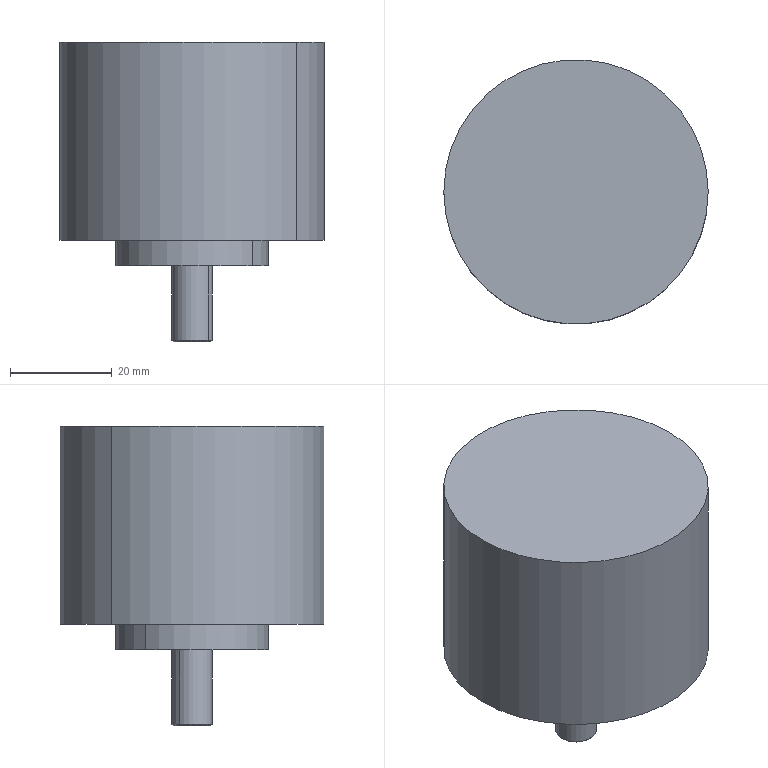Component | SolidWorks | LD101-02-RotaryEncoder-0002-2-2 | 1 solid | 24 faces | box 52 x 52 x 59 mm | volume 86983 mm3 | cylinder 12 | cone 8 | plane 4 | commonest cylinder face diameters 2.5 x6 8 x2 30 x2 52 x2 | material AL6061
STEP:
#1=COLOUR_RGB('',0.7922,0.8196,0.9333);
#2=FILL_AREA_STYLE_COLOUR('',#1);
#3=FILL_AREA_STYLE('',(#2));
#4=SURFACE_STYLE_FILL_AREA(#3);
#5=SURFACE_SIDE_STYLE('',(#4));
#6=SURFACE_STYLE_USAGE(.BOTH.,#5);
#7=PRESENTATION_STYLE_ASSIGNMENT((#6));
#8=CARTESIAN_POINT('',(5.132,-7.919,13.573));
#9=VERTEX_POINT('',#8);
#10=CARTESIAN_POINT('',(5.054,-7.859,13.573));
#11=VERTEX_POINT('',#10);
#12=CARTESIAN_POINT('',(5.093,-7.889,13.573));
#13=DIRECTION('',(0.,0.,-1.));
#14=DIRECTION('',(-0.7932,0.609,0.));
#15=AXIS2_PLACEMENT_3D('',#12,#13,#14);
#16=CIRCLE('',#15,0.04921);
#17=EDGE_CURVE('',#9,#11,#16,.T.);
#18=ORIENTED_EDGE('',*,*,#17,.F.);
#19=CARTESIAN_POINT('',(5.132,-7.919,13.238));
#20=VERTEX_POINT('',#19);
#21=CARTESIAN_POINT('',(5.132,-7.919,13.238));
#22=DIRECTION('',(0.,0.,-1.));
#23=VECTOR('',#22,39.37);
#24=LINE('',#21,#23);
#25=EDGE_CURVE('',#9,#20,#24,.T.);
#26=ORIENTED_EDGE('',*,*,#25,.T.);
#27=CARTESIAN_POINT('',(5.054,-7.859,13.238));
#28=VERTEX_POINT('',#27);
#29=CARTESIAN_POINT('',(5.093,-7.889,13.238));
#30=DIRECTION('',(0.,0.,-1.));
#31=DIRECTION('',(-0.7932,0.609,0.));
#32=AXIS2_PLACEMENT_3D('',#29,#30,#31);
#33=CIRCLE('',#32,0.04921);
#34=EDGE_CURVE('',#20,#28,#33,.T.);
#35=ORIENTED_EDGE('',*,*,#34,.T.);
#36=CARTESIAN_POINT('',(5.054,-7.859,13.238));
#37=DIRECTION('',(0.,0.,-1.));
#38=VECTOR('',#37,39.37);
#39=LINE('',#36,#38);
#40=EDGE_CURVE('',#11,#28,#39,.T.);
#41=ORIENTED_EDGE('',*,*,#40,.F.);
#42=EDGE_LOOP('',(#18,#26,#35,#41));
#43=FACE_OUTER_BOUND('',#42,.T.);
#44=CARTESIAN_POINT('',(5.093,-7.889,13.238));
#45=DIRECTION('',(0.,0.,-1.));
#46=DIRECTION('',(-0.7932,0.609,0.));
#47=AXIS2_PLACEMENT_3D('',#44,#45,#46);
#48=CYLINDRICAL_SURFACE('',#47,0.04921);
#49=ADVANCED_FACE('',(#43),#48,.F.);
#50=CARTESIAN_POINT('',(5.093,-7.889,13.603));
#51=VERTEX_POINT('',#50);
#52=CARTESIAN_POINT('',(5.054,-7.859,13.573));
#53=DIRECTION('',(-0.6799,0.522,-0.515));
#54=VECTOR('',#53,39.37);
#55=LINE('',#52,#54);
#56=EDGE_CURVE('',#51,#11,#55,.T.);
#57=ORIENTED_EDGE('',*,*,#56,.F.);
#58=CARTESIAN_POINT('',(5.132,-7.919,13.573));
#59=DIRECTION('',(0.6799,-0.522,-0.515));
#60=VECTOR('',#59,39.37);
#61=LINE('',#58,#60);
#62=EDGE_CURVE('',#51,#9,#61,.T.);
#63=ORIENTED_EDGE('',*,*,#62,.T.);
#64=ORIENTED_EDGE('',*,*,#17,.T.);
#65=EDGE_LOOP('',(#57,#63,#64));
#66=FACE_OUTER_BOUND('',#65,.T.);
#67=CARTESIAN_POINT('',(5.093,-7.889,13.573));
#68=DIRECTION('',(0.,0.,-1.));
#69=DIRECTION('',(-0.7932,0.609,0.));
#70=AXIS2_PLACEMENT_3D('',#67,#68,#69);
#71=CONICAL_SURFACE('',#70,0.04921,1.03);
#72=ADVANCED_FACE('',(#66),#71,.F.);
#73=CARTESIAN_POINT('',(4.05,-7.088,13.573));
#74=VERTEX_POINT('',#73);
#75=CARTESIAN_POINT('',(3.972,-7.028,13.573));
#76=VERTEX_POINT('',#75);
#77=CARTESIAN_POINT('',(4.011,-7.058,13.573));
#78=DIRECTION('',(0.,0.,-1.));
#79=DIRECTION('',(-0.7932,0.609,0.));
#80=AXIS2_PLACEMENT_3D('',#77,#78,#79);
#81=CIRCLE('',#80,0.04921);
#82=EDGE_CURVE('',#74,#76,#81,.T.);
#83=ORIENTED_EDGE('',*,*,#82,.F.);
#84=CARTESIAN_POINT('',(4.05,-7.088,13.238));
#85=VERTEX_POINT('',#84);
#86=CARTESIAN_POINT('',(4.05,-7.088,13.238));
#87=DIRECTION('',(0.,0.,-1.));
#88=VECTOR('',#87,39.37);
#89=LINE('',#86,#88);
#90=EDGE_CURVE('',#74,#85,#89,.T.);
#91=ORIENTED_EDGE('',*,*,#90,.T.);
#92=CARTESIAN_POINT('',(3.972,-7.028,13.238));
#93=VERTEX_POINT('',#92);
#94=CARTESIAN_POINT('',(4.011,-7.058,13.238));
#95=DIRECTION('',(0.,0.,-1.));
#96=DIRECTION('',(-0.7932,0.609,0.));
#97=AXIS2_PLACEMENT_3D('',#94,#95,#96);
#98=CIRCLE('',#97,0.04921);
#99=EDGE_CURVE('',#85,#93,#98,.T.);
#100=ORIENTED_EDGE('',*,*,#99,.T.);
#101=CARTESIAN_POINT('',(3.972,-7.028,13.238));
#102=DIRECTION('',(0.,0.,-1.));
#103=VECTOR('',#102,39.37);
#104=LINE('',#101,#103);
#105=EDGE_CURVE('',#76,#93,#104,.T.);
#106=ORIENTED_EDGE('',*,*,#105,.F.);
#107=EDGE_LOOP('',(#83,#91,#100,#106));
#108=FACE_OUTER_BOUND('',#107,.T.);
#109=CARTESIAN_POINT('',(4.011,-7.058,13.238));
#110=DIRECTION('',(0.,0.,-1.));
#111=DIRECTION('',(-0.7932,0.609,0.));
#112=AXIS2_PLACEMENT_3D('',#109,#110,#111);
#113=CYLINDRICAL_SURFACE('',#112,0.04921);
#114=ADVANCED_FACE('',(#108),#113,.F.);
#115=CARTESIAN_POINT('',(4.011,-7.058,13.603));
#116=VERTEX_POINT('',#115);
#117=CARTESIAN_POINT('',(3.972,-7.028,13.573));
#118=DIRECTION('',(-0.6799,0.522,-0.515));
#119=VECTOR('',#118,39.37);
#120=LINE('',#117,#119);
#121=EDGE_CURVE('',#116,#76,#120,.T.);
#122=ORIENTED_EDGE('',*,*,#121,.F.);
#123=CARTESIAN_POINT('',(4.05,-7.088,13.573));
#124=DIRECTION('',(0.6799,-0.522,-0.515));
#125=VECTOR('',#124,39.37);
#126=LINE('',#123,#125);
#127=EDGE_CURVE('',#116,#74,#126,.T.);
#128=ORIENTED_EDGE('',*,*,#127,.T.);
#129=ORIENTED_EDGE('',*,*,#82,.T.);
#130=EDGE_LOOP('',(#122,#128,#129));
#131=FACE_OUTER_BOUND('',#130,.T.);
#132=CARTESIAN_POINT('',(4.011,-7.058,13.573));
#133=DIRECTION('',(0.,0.,-1.));
#134=DIRECTION('',(-0.7932,0.609,0.));
#135=AXIS2_PLACEMENT_3D('',#132,#133,#134);
#136=CONICAL_SURFACE('',#135,0.04921,1.03);
#137=ADVANCED_FACE('',(#131),#136,.F.);
#138=CARTESIAN_POINT('',(5.31,-6.567,13.573));
#139=VERTEX_POINT('',#138);
#140=CARTESIAN_POINT('',(5.232,-6.507,13.573));
#141=VERTEX_POINT('',#140);
#142=CARTESIAN_POINT('',(5.271,-6.537,13.573));
#143=DIRECTION('',(0.,0.,-1.));
#144=DIRECTION('',(-0.7932,0.609,0.));
#145=AXIS2_PLACEMENT_3D('',#142,#143,#144);
#146=CIRCLE('',#145,0.04921);
#147=EDGE_CURVE('',#139,#141,#146,.T.);
#148=ORIENTED_EDGE('',*,*,#147,.F.);
#149=CARTESIAN_POINT('',(5.31,-6.567,13.238));
#150=VERTEX_POINT('',#149);
#151=CARTESIAN_POINT('',(5.31,-6.567,13.238));
#152=DIRECTION('',(0.,0.,-1.));
#153=VECTOR('',#152,39.37);
#154=LINE('',#151,#153);
#155=EDGE_CURVE('',#139,#150,#154,.T.);
#156=ORIENTED_EDGE('',*,*,#155,.T.);
#157=CARTESIAN_POINT('',(5.232,-6.507,13.238));
#158=VERTEX_POINT('',#157);
#159=CARTESIAN_POINT('',(5.271,-6.537,13.238));
#160=DIRECTION('',(0.,0.,-1.));
#161=DIRECTION('',(-0.7932,0.609,0.));
#162=AXIS2_PLACEMENT_3D('',#159,#160,#161);
#163=CIRCLE('',#162,0.04921);
#164=EDGE_CURVE('',#150,#158,#163,.T.);
#165=ORIENTED_EDGE('',*,*,#164,.T.);
#166=CARTESIAN_POINT('',(5.232,-6.507,13.238));
#167=DIRECTION('',(0.,0.,-1.));
#168=VECTOR('',#167,39.37);
#169=LINE('',#166,#168);
#170=EDGE_CURVE('',#141,#158,#169,.T.);
#171=ORIENTED_EDGE('',*,*,#170,.F.);
#172=EDGE_LOOP('',(#148,#156,#165,#171));
#173=FACE_OUTER_BOUND('',#172,.T.);
#174=CARTESIAN_POINT('',(5.271,-6.537,13.238));
#175=DIRECTION('',(0.,0.,-1.));
#176=DIRECTION('',(-0.7932,0.609,0.));
#177=AXIS2_PLACEMENT_3D('',#174,#175,#176);
#178=CYLINDRICAL_SURFACE('',#177,0.04921);
#179=ADVANCED_FACE('',(#173),#178,.F.);
#180=CARTESIAN_POINT('',(5.271,-6.537,13.603));
#181=VERTEX_POINT('',#180);
#182=CARTESIAN_POINT('',(5.232,-6.507,13.573));
#183=DIRECTION('',(-0.6799,0.522,-0.515));
#184=VECTOR('',#183,39.37);
#185=LINE('',#182,#184);
#186=EDGE_CURVE('',#181,#141,#185,.T.);
#187=ORIENTED_EDGE('',*,*,#186,.F.);
#188=CARTESIAN_POINT('',(5.31,-6.567,13.573));
#189=DIRECTION('',(0.6799,-0.522,-0.515));
#190=VECTOR('',#189,39.37);
#191=LINE('',#188,#190);
#192=EDGE_CURVE('',#181,#139,#191,.T.);
#193=ORIENTED_EDGE('',*,*,#192,.T.);
#194=ORIENTED_EDGE('',*,*,#147,.T.);
#195=EDGE_LOOP('',(#187,#193,#194));
#196=FACE_OUTER_BOUND('',#195,.T.);
#197=CARTESIAN_POINT('',(5.271,-6.537,13.573));
#198=DIRECTION('',(0.,0.,-1.));
#199=DIRECTION('',(-0.7932,0.609,0.));
#200=AXIS2_PLACEMENT_3D('',#197,#198,#199);
#201=CONICAL_SURFACE('',#200,0.04921,1.03);
#202=ADVANCED_FACE('',(#196),#201,.F.);
#203=CARTESIAN_POINT('',(4.676,-7.073,12.451));
#204=VERTEX_POINT('',#203);
#205=CARTESIAN_POINT('',(4.907,-7.25,12.451));
#206=VERTEX_POINT('',#205);
#207=CARTESIAN_POINT('',(4.792,-7.161,12.451));
#208=DIRECTION('',(0.,0.,-1.));
#209=DIRECTION('',(-0.7932,0.609,0.));
#210=AXIS2_PLACEMENT_3D('',#207,#208,#209);
#211=CIRCLE('',#210,0.1457);
#212=EDGE_CURVE('',#204,#206,#211,.T.);
#213=ORIENTED_EDGE('',*,*,#212,.F.);
#214=CARTESIAN_POINT('',(4.667,-7.065,12.463));
#215=VERTEX_POINT('',#214);
#216=CARTESIAN_POINT('',(4.676,-7.073,12.451));
#217=DIRECTION('',(-0.5609,0.4306,0.7071));
#218=VECTOR('',#217,39.37);
#219=LINE('',#216,#218);
#220=EDGE_CURVE('',#204,#215,#219,.T.);
#221=ORIENTED_EDGE('',*,*,#220,.T.);
#222=CARTESIAN_POINT('',(4.917,-7.257,12.463));
#223=VERTEX_POINT('',#222);
#224=CARTESIAN_POINT('',(4.792,-7.161,12.463));
#225=DIRECTION('',(0.,0.,1.));
#226=DIRECTION('',(-0.7932,0.609,0.));
#227=AXIS2_PLACEMENT_3D('',#224,#225,#226);
#228=CIRCLE('',#227,0.1575);
#229=EDGE_CURVE('',#223,#215,#228,.T.);
#230=ORIENTED_EDGE('',*,*,#229,.F.);
#231=CARTESIAN_POINT('',(4.907,-7.25,12.451));
#232=DIRECTION('',(0.5609,-0.4306,0.7071));
#233=VECTOR('',#232,39.37);
#234=LINE('',#231,#233);
#235=EDGE_CURVE('',#206,#223,#234,.T.);
#236=ORIENTED_EDGE('',*,*,#235,.F.);
#237=EDGE_LOOP('',(#213,#221,#230,#236));
#238=FACE_OUTER_BOUND('',#237,.T.);
#239=CARTESIAN_POINT('',(4.792,-7.161,12.451));
#240=DIRECTION('',(0.,0.,1.));
#241=DIRECTION('',(0.7932,-0.609,0.));
#242=AXIS2_PLACEMENT_3D('',#239,#240,#241);
#243=CONICAL_SURFACE('',#242,0.1457,0.7854);
#244=ADVANCED_FACE('',(#238),#243,.T.);
#245=ORIENTED_EDGE('',*,*,#229,.T.);
#246=CARTESIAN_POINT('',(4.667,-7.065,13.042));
#247=VERTEX_POINT('',#246);
#248=CARTESIAN_POINT('',(4.667,-7.065,12.451));
#249=DIRECTION('',(0.,0.,1.));
#250=VECTOR('',#249,39.37);
#251=LINE('',#248,#250);
#252=EDGE_CURVE('',#215,#247,#251,.T.);
#253=ORIENTED_EDGE('',*,*,#252,.T.);
#254=CARTESIAN_POINT('',(4.917,-7.257,13.042));
#255=VERTEX_POINT('',#254);
#256=CARTESIAN_POINT('',(4.792,-7.161,13.042));
#257=DIRECTION('',(0.,0.,-1.));
#258=DIRECTION('',(-0.7932,0.609,0.));
#259=AXIS2_PLACEMENT_3D('',#256,#257,#258);
#260=CIRCLE('',#259,0.1575);
#261=EDGE_CURVE('',#247,#255,#260,.T.);
#262=ORIENTED_EDGE('',*,*,#261,.T.);
#263=CARTESIAN_POINT('',(4.917,-7.257,12.451));
#264=DIRECTION('',(0.,0.,1.));
#265=VECTOR('',#264,39.37);
#266=LINE('',#263,#265);
#267=EDGE_CURVE('',#223,#255,#266,.T.);
#268=ORIENTED_EDGE('',*,*,#267,.F.);
#269=EDGE_LOOP('',(#245,#253,#262,#268));
#270=FACE_OUTER_BOUND('',#269,.T.);
#271=CARTESIAN_POINT('',(4.792,-7.161,12.451));
#272=DIRECTION('',(0.,0.,1.));
#273=DIRECTION('',(0.7932,-0.609,0.));
#274=AXIS2_PLACEMENT_3D('',#271,#272,#273);
#275=CYLINDRICAL_SURFACE('',#274,0.1575);
#276=ADVANCED_FACE('',(#270),#275,.T.);
#277=CARTESIAN_POINT('',(4.323,-6.802,13.042));
#278=VERTEX_POINT('',#277);
#279=CARTESIAN_POINT('',(5.26,-7.521,13.042));
#280=VERTEX_POINT('',#279);
#281=CARTESIAN_POINT('',(4.792,-7.161,13.042));
#282=DIRECTION('',(0.,0.,-1.));
#283=DIRECTION('',(-0.7932,0.609,0.));
#284=AXIS2_PLACEMENT_3D('',#281,#282,#283);
#285=CIRCLE('',#284,0.5906);
#286=EDGE_CURVE('',#278,#280,#285,.T.);
#287=ORIENTED_EDGE('',*,*,#286,.F.);
#288=CARTESIAN_POINT('',(4.323,-6.802,13.238));
#289=VERTEX_POINT('',#288);
#290=CARTESIAN_POINT('',(4.323,-6.802,13.042));
#291=DIRECTION('',(0.,0.,1.));
#292=VECTOR('',#291,39.37);
#293=LINE('',#290,#292);
#294=EDGE_CURVE('',#278,#289,#293,.T.);
#295=ORIENTED_EDGE('',*,*,#294,.T.);
#296=CARTESIAN_POINT('',(5.26,-7.521,13.238));
#297=VERTEX_POINT('',#296);
#298=CARTESIAN_POINT('',(4.792,-7.161,13.238));
#299=DIRECTION('',(0.,0.,-1.));
#300=DIRECTION('',(-0.7932,0.609,0.));
#301=AXIS2_PLACEMENT_3D('',#298,#299,#300);
#302=CIRCLE('',#301,0.5906);
#303=EDGE_CURVE('',#289,#297,#302,.T.);
#304=ORIENTED_EDGE('',*,*,#303,.T.);
#305=CARTESIAN_POINT('',(5.26,-7.521,13.042));
#306=DIRECTION('',(0.,0.,1.));
#307=VECTOR('',#306,39.37);
#308=LINE('',#305,#307);
#309=EDGE_CURVE('',#280,#297,#308,.T.);
#310=ORIENTED_EDGE('',*,*,#309,.F.);
#311=EDGE_LOOP('',(#287,#295,#304,#310));
#312=FACE_OUTER_BOUND('',#311,.T.);
#313=CARTESIAN_POINT('',(4.792,-7.161,13.042));
#314=DIRECTION('',(0.,0.,1.));
#315=DIRECTION('',(0.7932,-0.609,0.));
#316=AXIS2_PLACEMENT_3D('',#313,#314,#315);
#317=CYLINDRICAL_SURFACE('',#316,0.5906);
#318=ADVANCED_FACE('',(#312),#317,.T.);
#319=CARTESIAN_POINT('',(3.98,-6.538,14.774));
#320=VERTEX_POINT('',#319);
#321=CARTESIAN_POINT('',(5.604,-7.785,14.774));
#322=VERTEX_POINT('',#321);
#323=CARTESIAN_POINT('',(4.792,-7.161,14.774));
#324=DIRECTION('',(0.,0.,-1.));
#325=DIRECTION('',(-0.7932,0.609,0.));
#326=AXIS2_PLACEMENT_3D('',#323,#324,#325);
#327=CIRCLE('',#326,1.024);
#328=EDGE_CURVE('',#320,#322,#327,.T.);
#329=ORIENTED_EDGE('',*,*,#328,.T.);
#330=CARTESIAN_POINT('',(5.604,-7.785,13.238));
#331=VERTEX_POINT('',#330);
#332=CARTESIAN_POINT('',(5.604,-7.785,14.774));
#333=DIRECTION('',(0.,0.,-1.));
#334=VECTOR('',#333,39.37);
#335=LINE('',#332,#334);
#336=EDGE_CURVE('',#322,#331,#335,.T.);
#337=ORIENTED_EDGE('',*,*,#336,.T.);
#338=CARTESIAN_POINT('',(3.98,-6.538,13.238));
#339=VERTEX_POINT('',#338);
#340=CARTESIAN_POINT('',(4.792,-7.161,13.238));
#341=DIRECTION('',(0.,0.,-1.));
#342=DIRECTION('',(-0.7932,0.609,0.));
#343=AXIS2_PLACEMENT_3D('',#340,#341,#342);
#344=CIRCLE('',#343,1.024);
#345=EDGE_CURVE('',#339,#331,#344,.T.);
#346=ORIENTED_EDGE('',*,*,#345,.F.);
#347=CARTESIAN_POINT('',(3.98,-6.538,14.774));
#348=DIRECTION('',(0.,0.,-1.));
#349=VECTOR('',#348,39.37);
#350=LINE('',#347,#349);
#351=EDGE_CURVE('',#320,#339,#350,.T.);
#352=ORIENTED_EDGE('',*,*,#351,.F.);
#353=EDGE_LOOP('',(#329,#337,#346,#352));
#354=FACE_OUTER_BOUND('',#353,.T.);
#355=CARTESIAN_POINT('',(4.792,-7.161,14.774));
#356=DIRECTION('',(0.,0.,-1.));
#357=DIRECTION('',(-0.7932,0.609,0.));
#358=AXIS2_PLACEMENT_3D('',#355,#356,#357);
#359=CYLINDRICAL_SURFACE('',#358,1.024);
#360=ADVANCED_FACE('',(#354),#359,.T.);
#361=CARTESIAN_POINT('',(4.792,-7.161,13.042));
#362=DIRECTION('',(0.,0.,-1.));
#363=DIRECTION('',(-0.7932,0.609,0.));
#364=AXIS2_PLACEMENT_3D('',#361,#362,#363);
#365=CIRCLE('',#364,0.5906);
#366=EDGE_CURVE('',#280,#278,#365,.T.);
#367=ORIENTED_EDGE('',*,*,#366,.T.);
#368=ORIENTED_EDGE('',*,*,#286,.T.);
#369=EDGE_LOOP('',(#367,#368));
#370=FACE_OUTER_BOUND('',#369,.T.);
#371=CARTESIAN_POINT('',(4.792,-7.161,13.042));
#372=DIRECTION('',(0.,0.,-1.));
#373=DIRECTION('',(-0.7932,0.609,0.));
#374=AXIS2_PLACEMENT_3D('',#371,#372,#373);
#375=CIRCLE('',#374,0.1575);
#376=EDGE_CURVE('',#255,#247,#375,.T.);
#377=ORIENTED_EDGE('',*,*,#376,.F.);
#378=ORIENTED_EDGE('',*,*,#261,.F.);
#379=EDGE_LOOP('',(#377,#378));
#380=FACE_BOUND('',#379,.T.);
#381=CARTESIAN_POINT('',(4.792,-7.161,13.042));
#382=DIRECTION('',(0.,0.,-1.));
#383=DIRECTION('',(-0.7932,0.609,0.));
#384=AXIS2_PLACEMENT_3D('',#381,#382,#383);
#385=PLANE('',#384);
#386=ADVANCED_FACE('',(#370,#380),#385,.T.);
#387=CARTESIAN_POINT('',(5.093,-7.889,13.238));
#388=DIRECTION('',(0.,0.,-1.));
#389=DIRECTION('',(-0.7932,0.609,0.));
#390=AXIS2_PLACEMENT_3D('',#387,#388,#389);
#391=CIRCLE('',#390,0.04921);
#392=EDGE_CURVE('',#28,#20,#391,.T.);
#393=ORIENTED_EDGE('',*,*,#392,.F.);
#394=ORIENTED_EDGE('',*,*,#34,.F.);
#395=EDGE_LOOP('',(#393,#394));
#396=FACE_BOUND('',#395,.T.);
#397=CARTESIAN_POINT('',(4.011,-7.058,13.238));
#398=DIRECTION('',(0.,0.,-1.));
#399=DIRECTION('',(-0.7932,0.609,0.));
#400=AXIS2_PLACEMENT_3D('',#397,#398,#399);
#401=CIRCLE('',#400,0.04921);
#402=EDGE_CURVE('',#93,#85,#401,.T.);
#403=ORIENTED_EDGE('',*,*,#402,.F.);
#404=ORIENTED_EDGE('',*,*,#99,.F.);
#405=EDGE_LOOP('',(#403,#404));
#406=FACE_BOUND('',#405,.T.);
#407=CARTESIAN_POINT('',(5.271,-6.537,13.238));
#408=DIRECTION('',(0.,0.,-1.));
#409=DIRECTION('',(-0.7932,0.609,0.));
#410=AXIS2_PLACEMENT_3D('',#407,#408,#409);
#411=CIRCLE('',#410,0.04921);
#412=EDGE_CURVE('',#158,#150,#411,.T.);
#413=ORIENTED_EDGE('',*,*,#412,.F.);
#414=ORIENTED_EDGE('',*,*,#164,.F.);
#415=EDGE_LOOP('',(#413,#414));
#416=FACE_BOUND('',#415,.T.);
#417=ORIENTED_EDGE('',*,*,#345,.T.);
#418=CARTESIAN_POINT('',(4.792,-7.161,13.238));
#419=DIRECTION('',(0.,0.,-1.));
#420=DIRECTION('',(-0.7932,0.609,0.));
#421=AXIS2_PLACEMENT_3D('',#418,#419,#420);
#422=CIRCLE('',#421,1.024);
#423=EDGE_CURVE('',#331,#339,#422,.T.);
#424=ORIENTED_EDGE('',*,*,#423,.T.);
#425=EDGE_LOOP('',(#417,#424));
#426=FACE_OUTER_BOUND('',#425,.T.);
#427=CARTESIAN_POINT('',(4.792,-7.161,13.238));
#428=DIRECTION('',(0.,0.,-1.));
#429=DIRECTION('',(-0.7932,0.609,0.));
#430=AXIS2_PLACEMENT_3D('',#427,#428,#429);
#431=CIRCLE('',#430,0.5906);
#432=EDGE_CURVE('',#297,#289,#431,.T.);
#433=ORIENTED_EDGE('',*,*,#432,.F.);
#434=ORIENTED_EDGE('',*,*,#303,.F.);
#435=EDGE_LOOP('',(#433,#434));
#436=FACE_BOUND('',#435,.T.);
#437=CARTESIAN_POINT('',(4.792,-7.161,13.238));
#438=DIRECTION('',(0.,0.,-1.));
#439=DIRECTION('',(-0.7932,0.609,0.));
#440=AXIS2_PLACEMENT_3D('',#437,#438,#439);
#441=PLANE('',#440);
#442=ADVANCED_FACE('',(#396,#406,#416,#426,#436),#441,.T.);
#443=ORIENTED_EDGE('',*,*,#336,.F.);
#444=CARTESIAN_POINT('',(4.792,-7.161,14.774));
#445=DIRECTION('',(0.,0.,-1.));
#446=DIRECTION('',(-0.7932,0.609,0.));
#447=AXIS2_PLACEMENT_3D('',#444,#445,#446);
#448=CIRCLE('',#447,1.024);
#449=EDGE_CURVE('',#322,#320,#448,.T.);
#450=ORIENTED_EDGE('',*,*,#449,.T.);
#451=ORIENTED_EDGE('',*,*,#351,.T.);
#452=ORIENTED_EDGE('',*,*,#423,.F.);
#453=EDGE_LOOP('',(#443,#450,#451,#452));
#454=FACE_OUTER_BOUND('',#453,.T.);
#455=CARTESIAN_POINT('',(4.792,-7.161,14.774));
#456=DIRECTION('',(0.,0.,-1.));
#457=DIRECTION('',(-0.7932,0.609,0.));
#458=AXIS2_PLACEMENT_3D('',#455,#456,#457);
#459=CYLINDRICAL_SURFACE('',#458,1.024);
#460=ADVANCED_FACE('',(#454),#459,.T.);
#461=ORIENTED_EDGE('',*,*,#328,.F.);
#462=ORIENTED_EDGE('',*,*,#449,.F.);
#463=EDGE_LOOP('',(#461,#462));
#464=FACE_OUTER_BOUND('',#463,.T.);
#465=CARTESIAN_POINT('',(4.792,-7.161,14.774));
#466=DIRECTION('',(0.,0.,-1.));
#467=DIRECTION('',(-0.7932,0.609,0.));
#468=AXIS2_PLACEMENT_3D('',#465,#466,#467);
#469=PLANE('',#468);
#470=ADVANCED_FACE('',(#464),#469,.F.);
#471=ORIENTED_EDGE('',*,*,#294,.F.);
#472=ORIENTED_EDGE('',*,*,#366,.F.);
#473=ORIENTED_EDGE('',*,*,#309,.T.);
#474=ORIENTED_EDGE('',*,*,#432,.T.);
#475=EDGE_LOOP('',(#471,#472,#473,#474));
#476=FACE_OUTER_BOUND('',#475,.T.);
#477=CARTESIAN_POINT('',(4.792,-7.161,13.042));
#478=DIRECTION('',(0.,0.,1.));
#479=DIRECTION('',(0.7932,-0.609,0.));
#480=AXIS2_PLACEMENT_3D('',#477,#478,#479);
#481=CYLINDRICAL_SURFACE('',#480,0.5906);
#482=ADVANCED_FACE('',(#476),#481,.T.);
#483=ORIENTED_EDGE('',*,*,#252,.F.);
#484=CARTESIAN_POINT('',(4.792,-7.161,12.463));
#485=DIRECTION('',(0.,0.,1.));
#486=DIRECTION('',(-0.7932,0.609,0.));
#487=AXIS2_PLACEMENT_3D('',#484,#485,#486);
#488=CIRCLE('',#487,0.1575);
#489=EDGE_CURVE('',#215,#223,#488,.T.);
#490=ORIENTED_EDGE('',*,*,#489,.T.);
#491=ORIENTED_EDGE('',*,*,#267,.T.);
#492=ORIENTED_EDGE('',*,*,#376,.T.);
#493=EDGE_LOOP('',(#483,#490,#491,#492));
#494=FACE_OUTER_BOUND('',#493,.T.);
#495=CARTESIAN_POINT('',(4.792,-7.161,12.451));
#496=DIRECTION('',(0.,0.,1.));
#497=DIRECTION('',(0.7932,-0.609,0.));
#498=AXIS2_PLACEMENT_3D('',#495,#496,#497);
#499=CYLINDRICAL_SURFACE('',#498,0.1575);
#500=ADVANCED_FACE('',(#494),#499,.T.);
#501=CARTESIAN_POINT('',(4.792,-7.161,12.451));
#502=DIRECTION('',(0.,0.,-1.));
#503=DIRECTION('',(-0.7932,0.609,0.));
#504=AXIS2_PLACEMENT_3D('',#501,#502,#503);
#505=CIRCLE('',#504,0.1457);
#506=EDGE_CURVE('',#206,#204,#505,.T.);
#507=ORIENTED_EDGE('',*,*,#506,.T.);
#508=ORIENTED_EDGE('',*,*,#212,.T.);
#509=EDGE_LOOP('',(#507,#508));
#510=FACE_OUTER_BOUND('',#509,.T.);
#511=CARTESIAN_POINT('',(4.792,-7.161,12.451));
#512=DIRECTION('',(0.,0.,-1.));
#513=DIRECTION('',(-0.7932,0.609,0.));
#514=AXIS2_PLACEMENT_3D('',#511,#512,#513);
#515=PLANE('',#514);
#516=ADVANCED_FACE('',(#510),#515,.T.);
#517=ORIENTED_EDGE('',*,*,#220,.F.);
#518=ORIENTED_EDGE('',*,*,#506,.F.);
#519=ORIENTED_EDGE('',*,*,#235,.T.);
#520=ORIENTED_EDGE('',*,*,#489,.F.);
#521=EDGE_LOOP('',(#517,#518,#519,#520));
#522=FACE_OUTER_BOUND('',#521,.T.);
#523=CARTESIAN_POINT('',(4.792,-7.161,12.451));
#524=DIRECTION('',(0.,0.,1.));
#525=DIRECTION('',(0.7932,-0.609,0.));
#526=AXIS2_PLACEMENT_3D('',#523,#524,#525);
#527=CONICAL_SURFACE('',#526,0.1457,0.7854);
#528=ADVANCED_FACE('',(#522),#527,.T.);
#529=ORIENTED_EDGE('',*,*,#192,.F.);
#530=ORIENTED_EDGE('',*,*,#186,.T.);
#531=CARTESIAN_POINT('',(5.271,-6.537,13.573));
#532=DIRECTION('',(0.,0.,-1.));
#533=DIRECTION('',(-0.7932,0.609,0.));
#534=AXIS2_PLACEMENT_3D('',#531,#532,#533);
#535=CIRCLE('',#534,0.04921);
#536=EDGE_CURVE('',#141,#139,#535,.T.);
#537=ORIENTED_EDGE('',*,*,#536,.T.);
#538=EDGE_LOOP('',(#529,#530,#537));
#539=FACE_OUTER_BOUND('',#538,.T.);
#540=CARTESIAN_POINT('',(5.271,-6.537,13.573));
#541=DIRECTION('',(0.,0.,-1.));
#542=DIRECTION('',(-0.7932,0.609,0.));
#543=AXIS2_PLACEMENT_3D('',#540,#541,#542);
#544=CONICAL_SURFACE('',#543,0.04921,1.03);
#545=ADVANCED_FACE('',(#539),#544,.F.);
#546=ORIENTED_EDGE('',*,*,#155,.F.);
#547=ORIENTED_EDGE('',*,*,#536,.F.);
#548=ORIENTED_EDGE('',*,*,#170,.T.);
#549=ORIENTED_EDGE('',*,*,#412,.T.);
#550=EDGE_LOOP('',(#546,#547,#548,#549));
#551=FACE_OUTER_BOUND('',#550,.T.);
#552=CARTESIAN_POINT('',(5.271,-6.537,13.238));
#553=DIRECTION('',(0.,0.,-1.));
#554=DIRECTION('',(-0.7932,0.609,0.));
#555=AXIS2_PLACEMENT_3D('',#552,#553,#554);
#556=CYLINDRICAL_SURFACE('',#555,0.04921);
#557=ADVANCED_FACE('',(#551),#556,.F.);
#558=ORIENTED_EDGE('',*,*,#127,.F.);
#559=ORIENTED_EDGE('',*,*,#121,.T.);
#560=CARTESIAN_POINT('',(4.011,-7.058,13.573));
#561=DIRECTION('',(0.,0.,-1.));
#562=DIRECTION('',(-0.7932,0.609,0.));
#563=AXIS2_PLACEMENT_3D('',#560,#561,#562);
#564=CIRCLE('',#563,0.04921);
#565=EDGE_CURVE('',#76,#74,#564,.T.);
#566=ORIENTED_EDGE('',*,*,#565,.T.);
#567=EDGE_LOOP('',(#558,#559,#566));
#568=FACE_OUTER_BOUND('',#567,.T.);
#569=CARTESIAN_POINT('',(4.011,-7.058,13.573));
#570=DIRECTION('',(0.,0.,-1.));
#571=DIRECTION('',(-0.7932,0.609,0.));
#572=AXIS2_PLACEMENT_3D('',#569,#570,#571);
#573=CONICAL_SURFACE('',#572,0.04921,1.03);
#574=ADVANCED_FACE('',(#568),#573,.F.);
#575=ORIENTED_EDGE('',*,*,#90,.F.);
#576=ORIENTED_EDGE('',*,*,#565,.F.);
#577=ORIENTED_EDGE('',*,*,#105,.T.);
#578=ORIENTED_EDGE('',*,*,#402,.T.);
#579=EDGE_LOOP('',(#575,#576,#577,#578));
#580=FACE_OUTER_BOUND('',#579,.T.);
#581=CARTESIAN_POINT('',(4.011,-7.058,13.238));
#582=DIRECTION('',(0.,0.,-1.));
#583=DIRECTION('',(-0.7932,0.609,0.));
#584=AXIS2_PLACEMENT_3D('',#581,#582,#583);
#585=CYLINDRICAL_SURFACE('',#584,0.04921);
#586=ADVANCED_FACE('',(#580),#585,.F.);
#587=ORIENTED_EDGE('',*,*,#62,.F.);
#588=ORIENTED_EDGE('',*,*,#56,.T.);
#589=CARTESIAN_POINT('',(5.093,-7.889,13.573));
#590=DIRECTION('',(0.,0.,-1.));
#591=DIRECTION('',(-0.7932,0.609,0.));
#592=AXIS2_PLACEMENT_3D('',#589,#590,#591);
#593=CIRCLE('',#592,0.04921);
#594=EDGE_CURVE('',#11,#9,#593,.T.);
#595=ORIENTED_EDGE('',*,*,#594,.T.);
#596=EDGE_LOOP('',(#587,#588,#595));
#597=FACE_OUTER_BOUND('',#596,.T.);
#598=CARTESIAN_POINT('',(5.093,-7.889,13.573));
#599=DIRECTION('',(0.,0.,-1.));
#600=DIRECTION('',(-0.7932,0.609,0.));
#601=AXIS2_PLACEMENT_3D('',#598,#599,#600);
#602=CONICAL_SURFACE('',#601,0.04921,1.03);
#603=ADVANCED_FACE('',(#597),#602,.F.);
#604=ORIENTED_EDGE('',*,*,#25,.F.);
#605=ORIENTED_EDGE('',*,*,#594,.F.);
#606=ORIENTED_EDGE('',*,*,#40,.T.);
#607=ORIENTED_EDGE('',*,*,#392,.T.);
#608=EDGE_LOOP('',(#604,#605,#606,#607));
#609=FACE_OUTER_BOUND('',#608,.T.);
#610=CARTESIAN_POINT('',(5.093,-7.889,13.238));
#611=DIRECTION('',(0.,0.,-1.));
#612=DIRECTION('',(-0.7932,0.609,0.));
#613=AXIS2_PLACEMENT_3D('',#610,#611,#612);
#614=CYLINDRICAL_SURFACE('',#613,0.04921);
#615=ADVANCED_FACE('',(#609),#614,.F.);
#616=CLOSED_SHELL('',(#49,#72,#114,#137,#179,#202,#244,#276,#318,#360,#386,#442,#460,#470,#482,#500,#516,#528,#545,#557,#574,#586,#603,#615));
#617=MANIFOLD_SOLID_BREP('',#616);
#618=STYLED_ITEM('',(#7),#617);
#619=PRESENTATION_LAYER_ASSIGNMENT('','',(#618));
#620=(LENGTH_UNIT()NAMED_UNIT(*)SI_UNIT($,.METRE.));
#621=LENGTH_MEASURE_WITH_UNIT(LENGTH_MEASURE(0.0254),#620);
#622=DIMENSIONAL_EXPONENTS(1.,0.,0.,0.,0.,0.,0.);
#623=(CONVERSION_BASED_UNIT('',#621)LENGTH_UNIT()NAMED_UNIT(#622));
#624=UNCERTAINTY_MEASURE_WITH_UNIT(LENGTH_MEASURE(0.00001),#623,'','');
#625=(NAMED_UNIT(*)PLANE_ANGLE_UNIT()SI_UNIT($,.RADIAN.));
#626=(NAMED_UNIT(*)SI_UNIT($,.STERADIAN.)SOLID_ANGLE_UNIT());
#627=(GEOMETRIC_REPRESENTATION_CONTEXT(3)GLOBAL_UNCERTAINTY_ASSIGNED_CONTEXT((#624))GLOBAL_UNIT_ASSIGNED_CONTEXT((#623,#625,#626))REPRESENTATION_CONTEXT('',''));
#628=MECHANICAL_DESIGN_GEOMETRIC_PRESENTATION_REPRESENTATION('',(#618),#627);
#629=CARTESIAN_POINT('',(0.,0.,0.));
#630=DIRECTION('',(0.,0.,1.));
#631=DIRECTION('',(1.,0.,0.));
#632=AXIS2_PLACEMENT_3D('',#629,#630,#631);
#633=(LENGTH_UNIT()NAMED_UNIT(*)SI_UNIT($,.METRE.));
#634=LENGTH_MEASURE_WITH_UNIT(LENGTH_MEASURE(0.0254),#633);
#635=DIMENSIONAL_EXPONENTS(1.,0.,0.,0.,0.,0.,0.);
#636=(CONVERSION_BASED_UNIT('',#634)LENGTH_UNIT()NAMED_UNIT(#635));
#637=UNCERTAINTY_MEASURE_WITH_UNIT(LENGTH_MEASURE(0.00001),#636,'','');
#638=(NAMED_UNIT(*)PLANE_ANGLE_UNIT()SI_UNIT($,.RADIAN.));
#639=(NAMED_UNIT(*)SI_UNIT($,.STERADIAN.)SOLID_ANGLE_UNIT());
#640=(GEOMETRIC_REPRESENTATION_CONTEXT(3)GLOBAL_UNCERTAINTY_ASSIGNED_CONTEXT((#637))GLOBAL_UNIT_ASSIGNED_CONTEXT((#636,#638,#639))REPRESENTATION_CONTEXT('',''));
#641=ADVANCED_BREP_SHAPE_REPRESENTATION('',(#617,#632),#640);